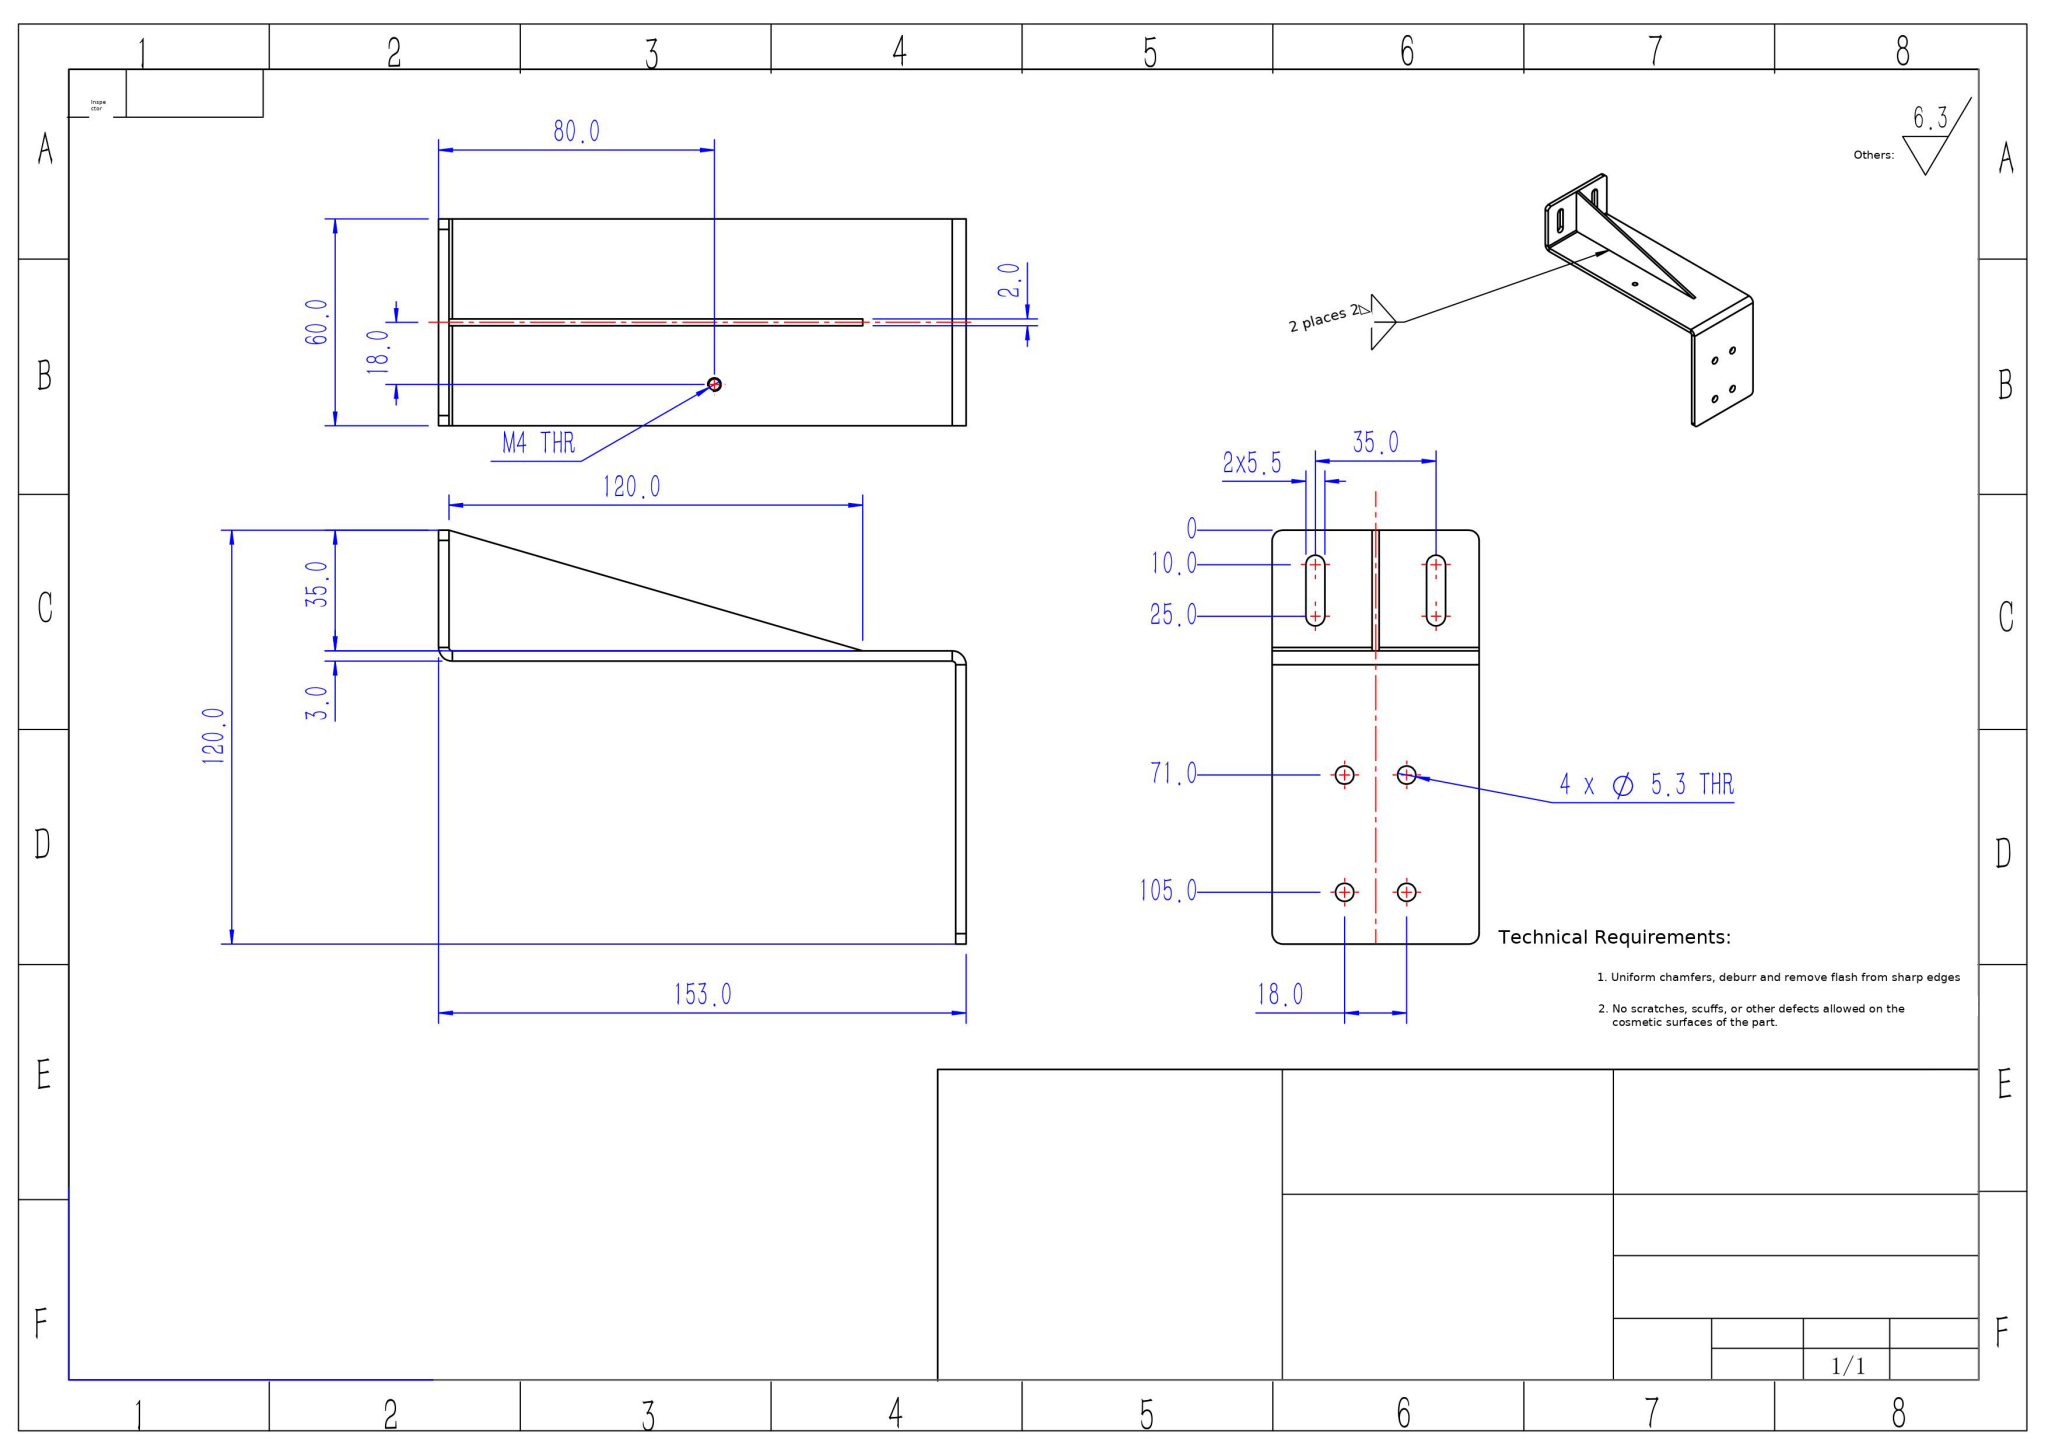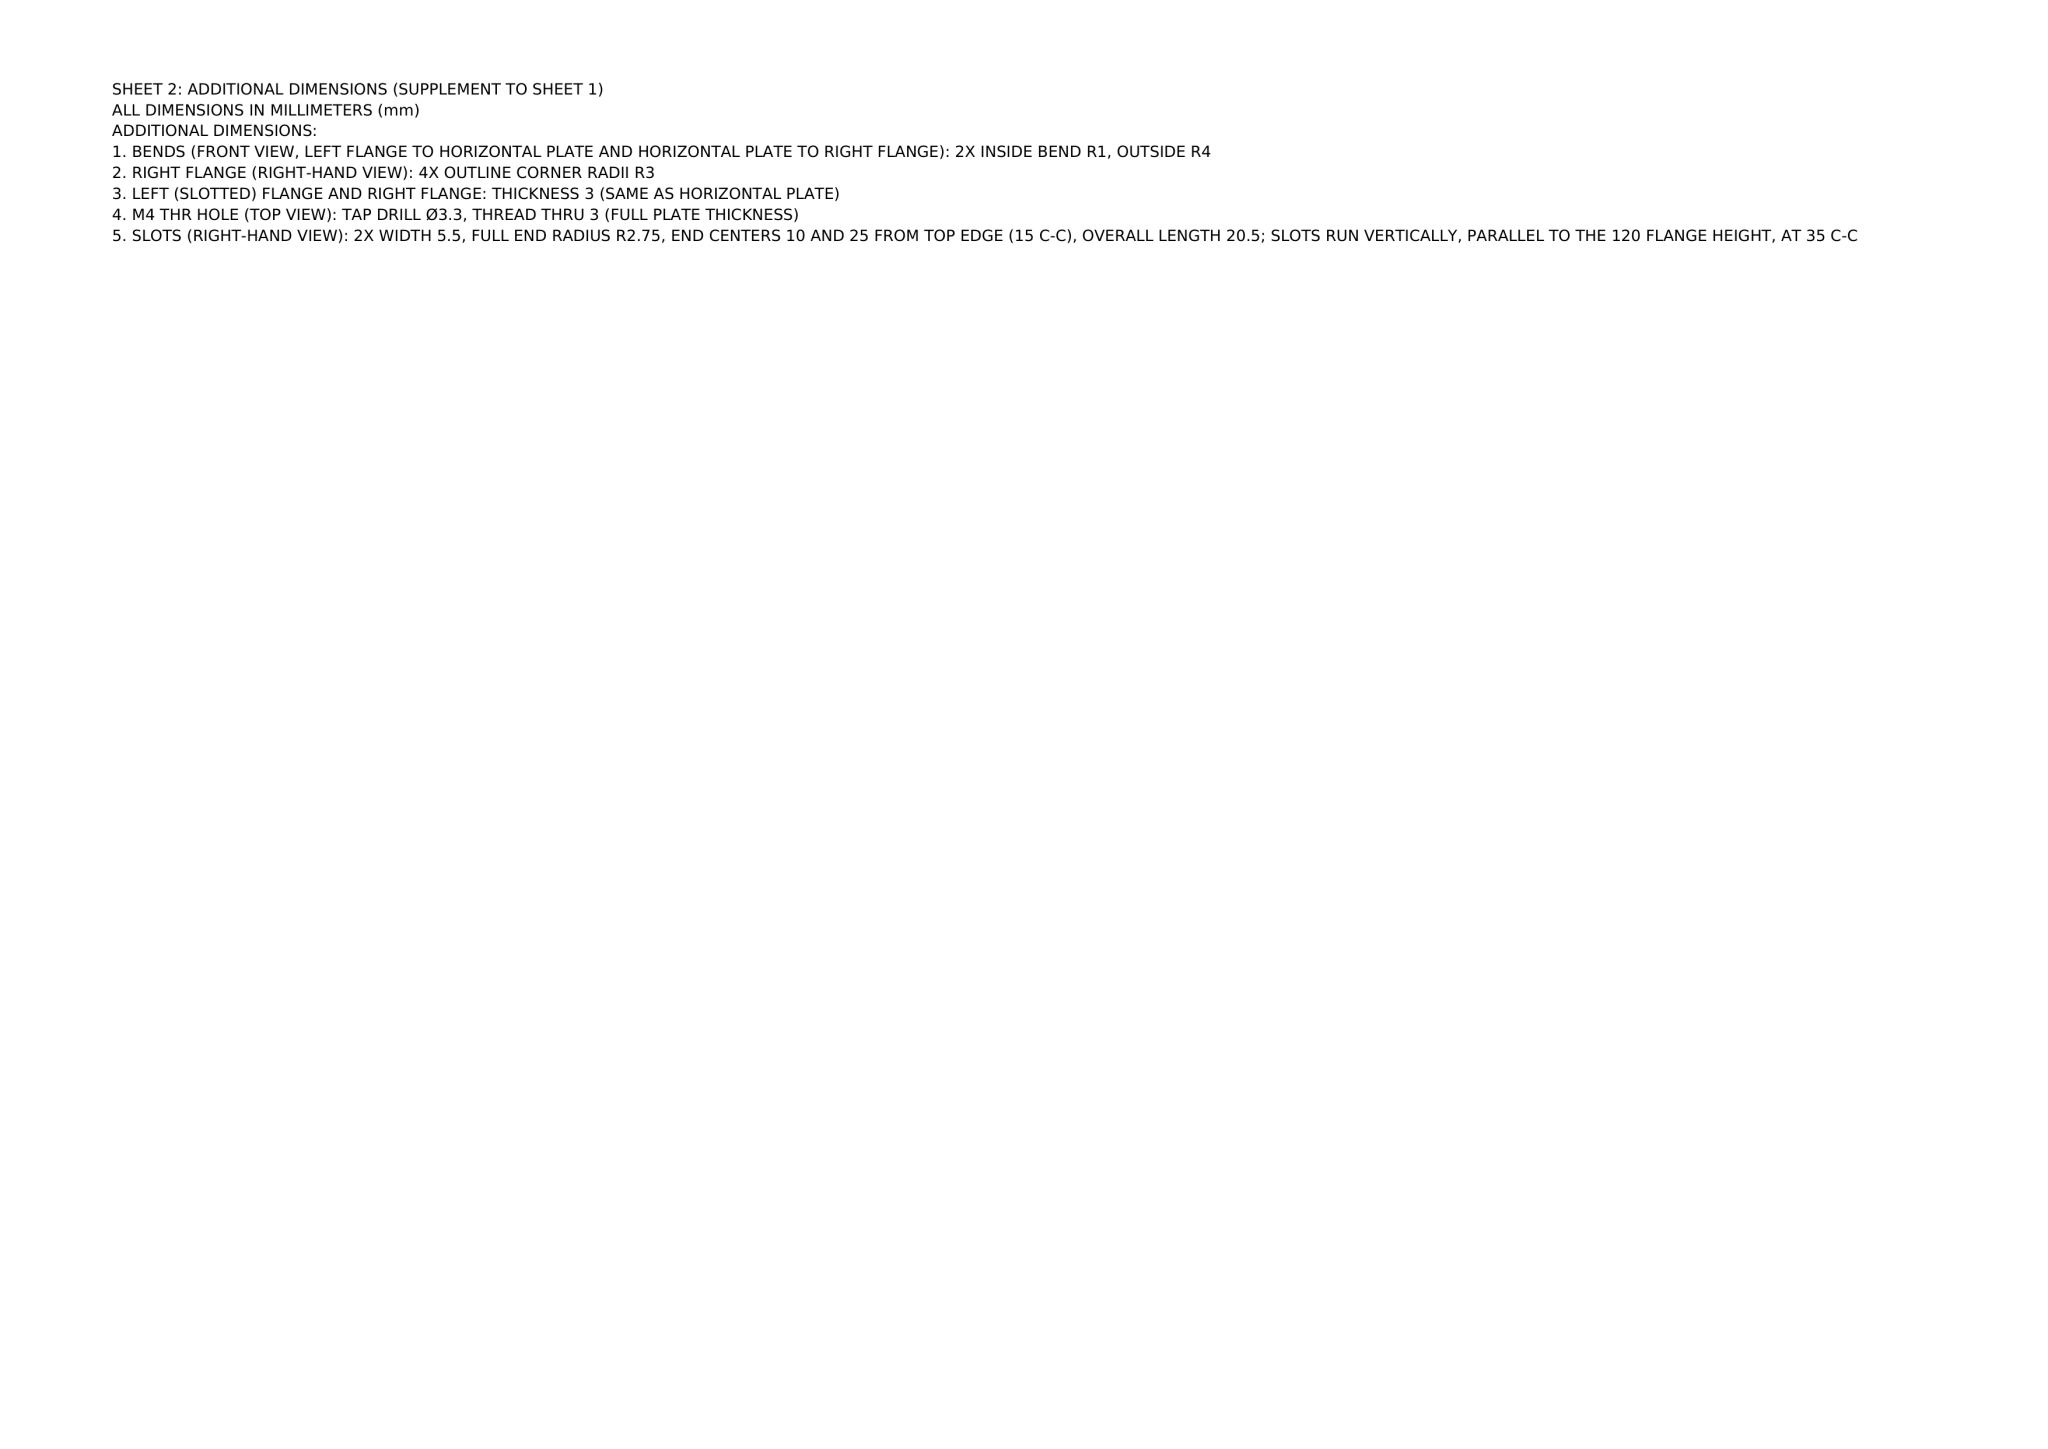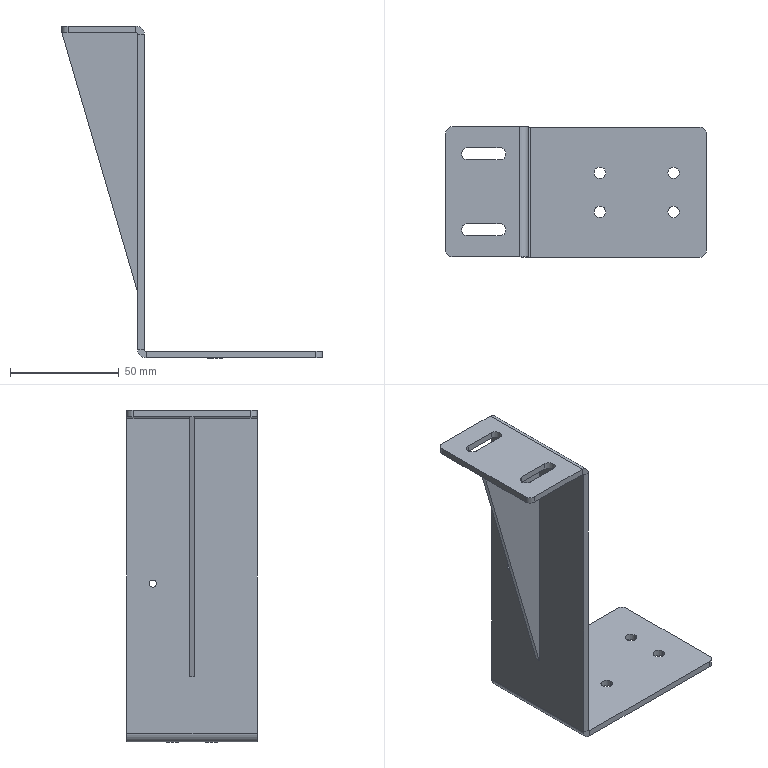Part | NX | mm | 1 solid | 51 faces | box 120 x 60 x 153 mm | volume 51462 mm3 | plane 26 | cylinder 25 | commonest cylinder face diameters 5.3 x8 5.5 x6 6 x4 2 x3 3.3 x2 8 x2